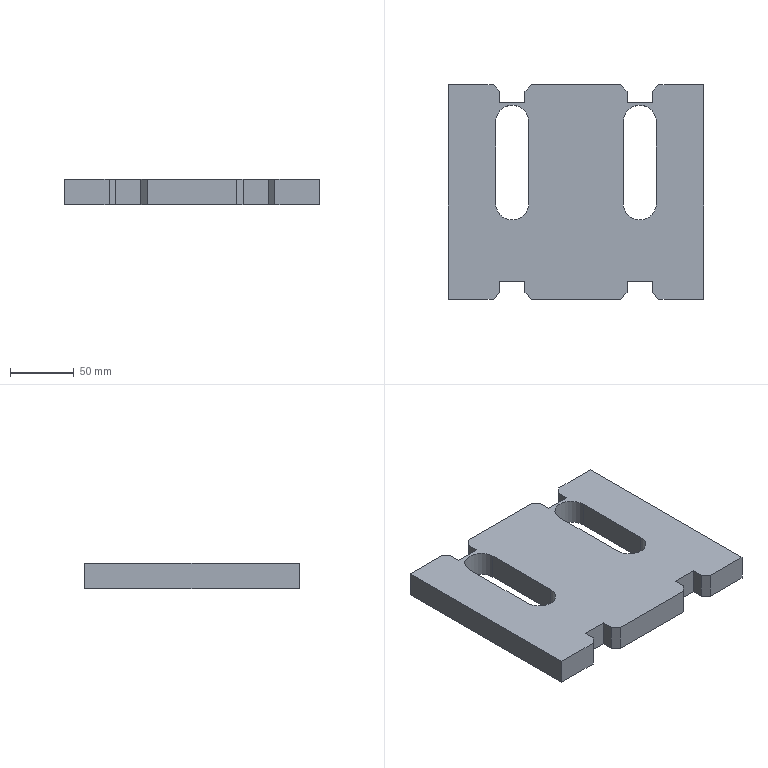Component | SolidWorks | NewTypeCurveBenderReinforcementSeatUpperWheelBox3-DoubleWheel-1 | 1 solid | 38 faces | box 200 x 168 x 20 mm | volume 559803 mm3 | plane 34 | cylinder 4 | commonest cylinder face diameters 26 x4
build123d program:
from build123d import *

# Parameters (mm, degrees)
SKETCH1_W           = 200
SKETCH1_H           = 168
BOSS_EXTRUDE1_DEPTH = 20
CUT_EXTRUDE1_DEPTH  = 20
SKETCH3_W           = 20
SKETCH3_H           = 28
CUT_EXTRUDE2_DEPTH  = 20
CHAMFER1_SIZE       = 5


with BuildPart() as part:
    # Sketch1 → Boss-Extrude1 (new body)
    with BuildSketch(Plane.XY):
        Rectangle(SKETCH1_W, SKETCH1_H)
    extrude(amount=BOSS_EXTRUDE1_DEPTH)

    # Sketch2 → Cut-Extrude1 (cut)
    with BuildSketch(Plane.XY.offset(20)):
        with BuildLine():
            Line((-37, 9), (-37, -55))
            ThreePointArc((-37, -55), (-50, -68), (-63, -55))
            Line((-63, -55), (-63, 9))
            ThreePointArc((-63, 9), (-50, 22), (-37, 9))
        make_face()
        with BuildLine():
            Line((37, 9), (37, -55))
            ThreePointArc((37, -55), (50, -68), (63, -55))
            Line((63, -55), (63, 9))
            ThreePointArc((63, 9), (50, 22), (37, 9))
        make_face()
    extrude(amount=-CUT_EXTRUDE1_DEPTH, mode=Mode.SUBTRACT)

    # Sketch3 → Cut-Extrude2 (cut)
    with BuildSketch(Plane.XY.offset(20)):
        with Locations((-50, 84)):
            Rectangle(SKETCH3_W, SKETCH3_H)
        with Locations((-50, -84)):
            Rectangle(SKETCH3_W, SKETCH3_H)
        with Locations((50, -84)):
            Rectangle(SKETCH3_W, SKETCH3_H)
        with Locations((50, 84)):
            Rectangle(SKETCH3_W, SKETCH3_H)
    extrude(amount=-CUT_EXTRUDE2_DEPTH, mode=Mode.SUBTRACT)

    # Chamfer1
    chamfer1_edges = [part.edges().sort_by_distance(p)[0] for p in [
        (60, 84, 10),
        (40, 84, 10),
        (60, -84, 10),
        (40, -84, 10),
        (-40, -84, 10),
        (-60, -84, 10),
        (-40, 84, 10),
        (-60, 84, 10),
    ]]
    chamfer(chamfer1_edges, length=CHAMFER1_SIZE)


solid = part.part

# Placed as in the assembly
solid = solid.moved(Location((0, -217, 59), (180, 0, 0)))